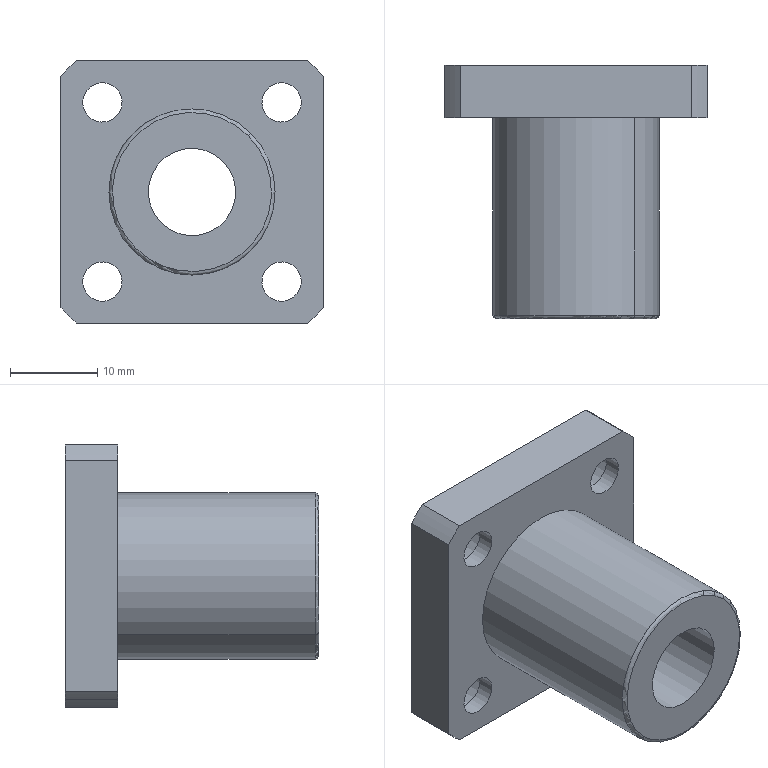Component | SolidWorks | LME13-d10.stp-1 | 1 solid | 38 faces | volume 8760 mm3 | cylinder 25 | plane 11 | torus 2 | commonest cylinder face diameters 7.5 x8 4.5 x8 40 x5 10 x2 19 x2